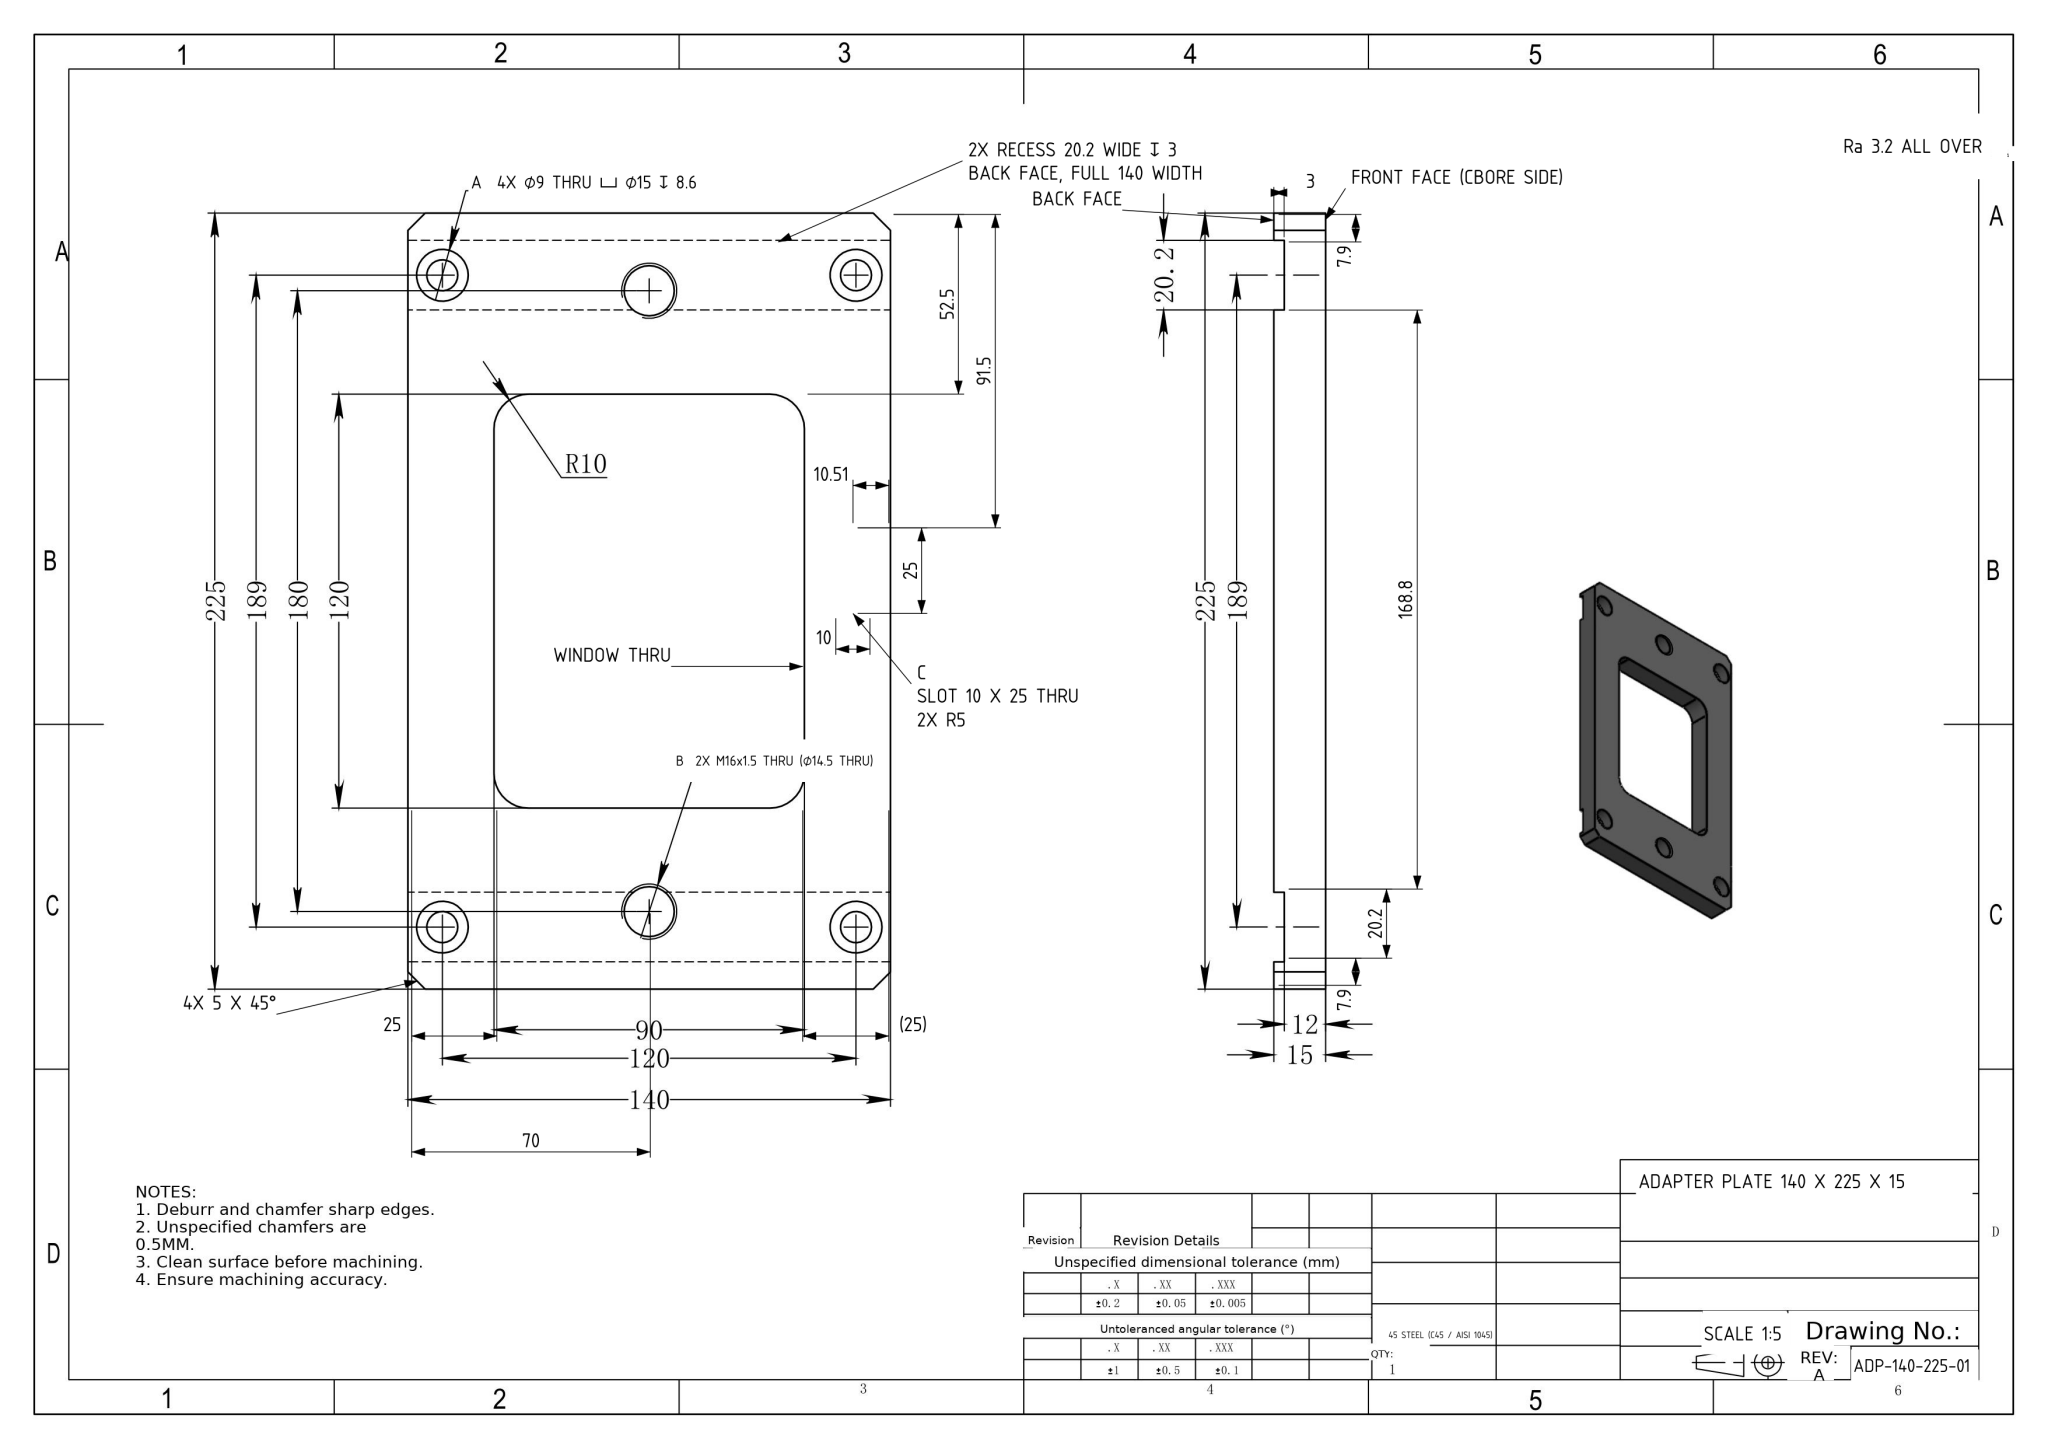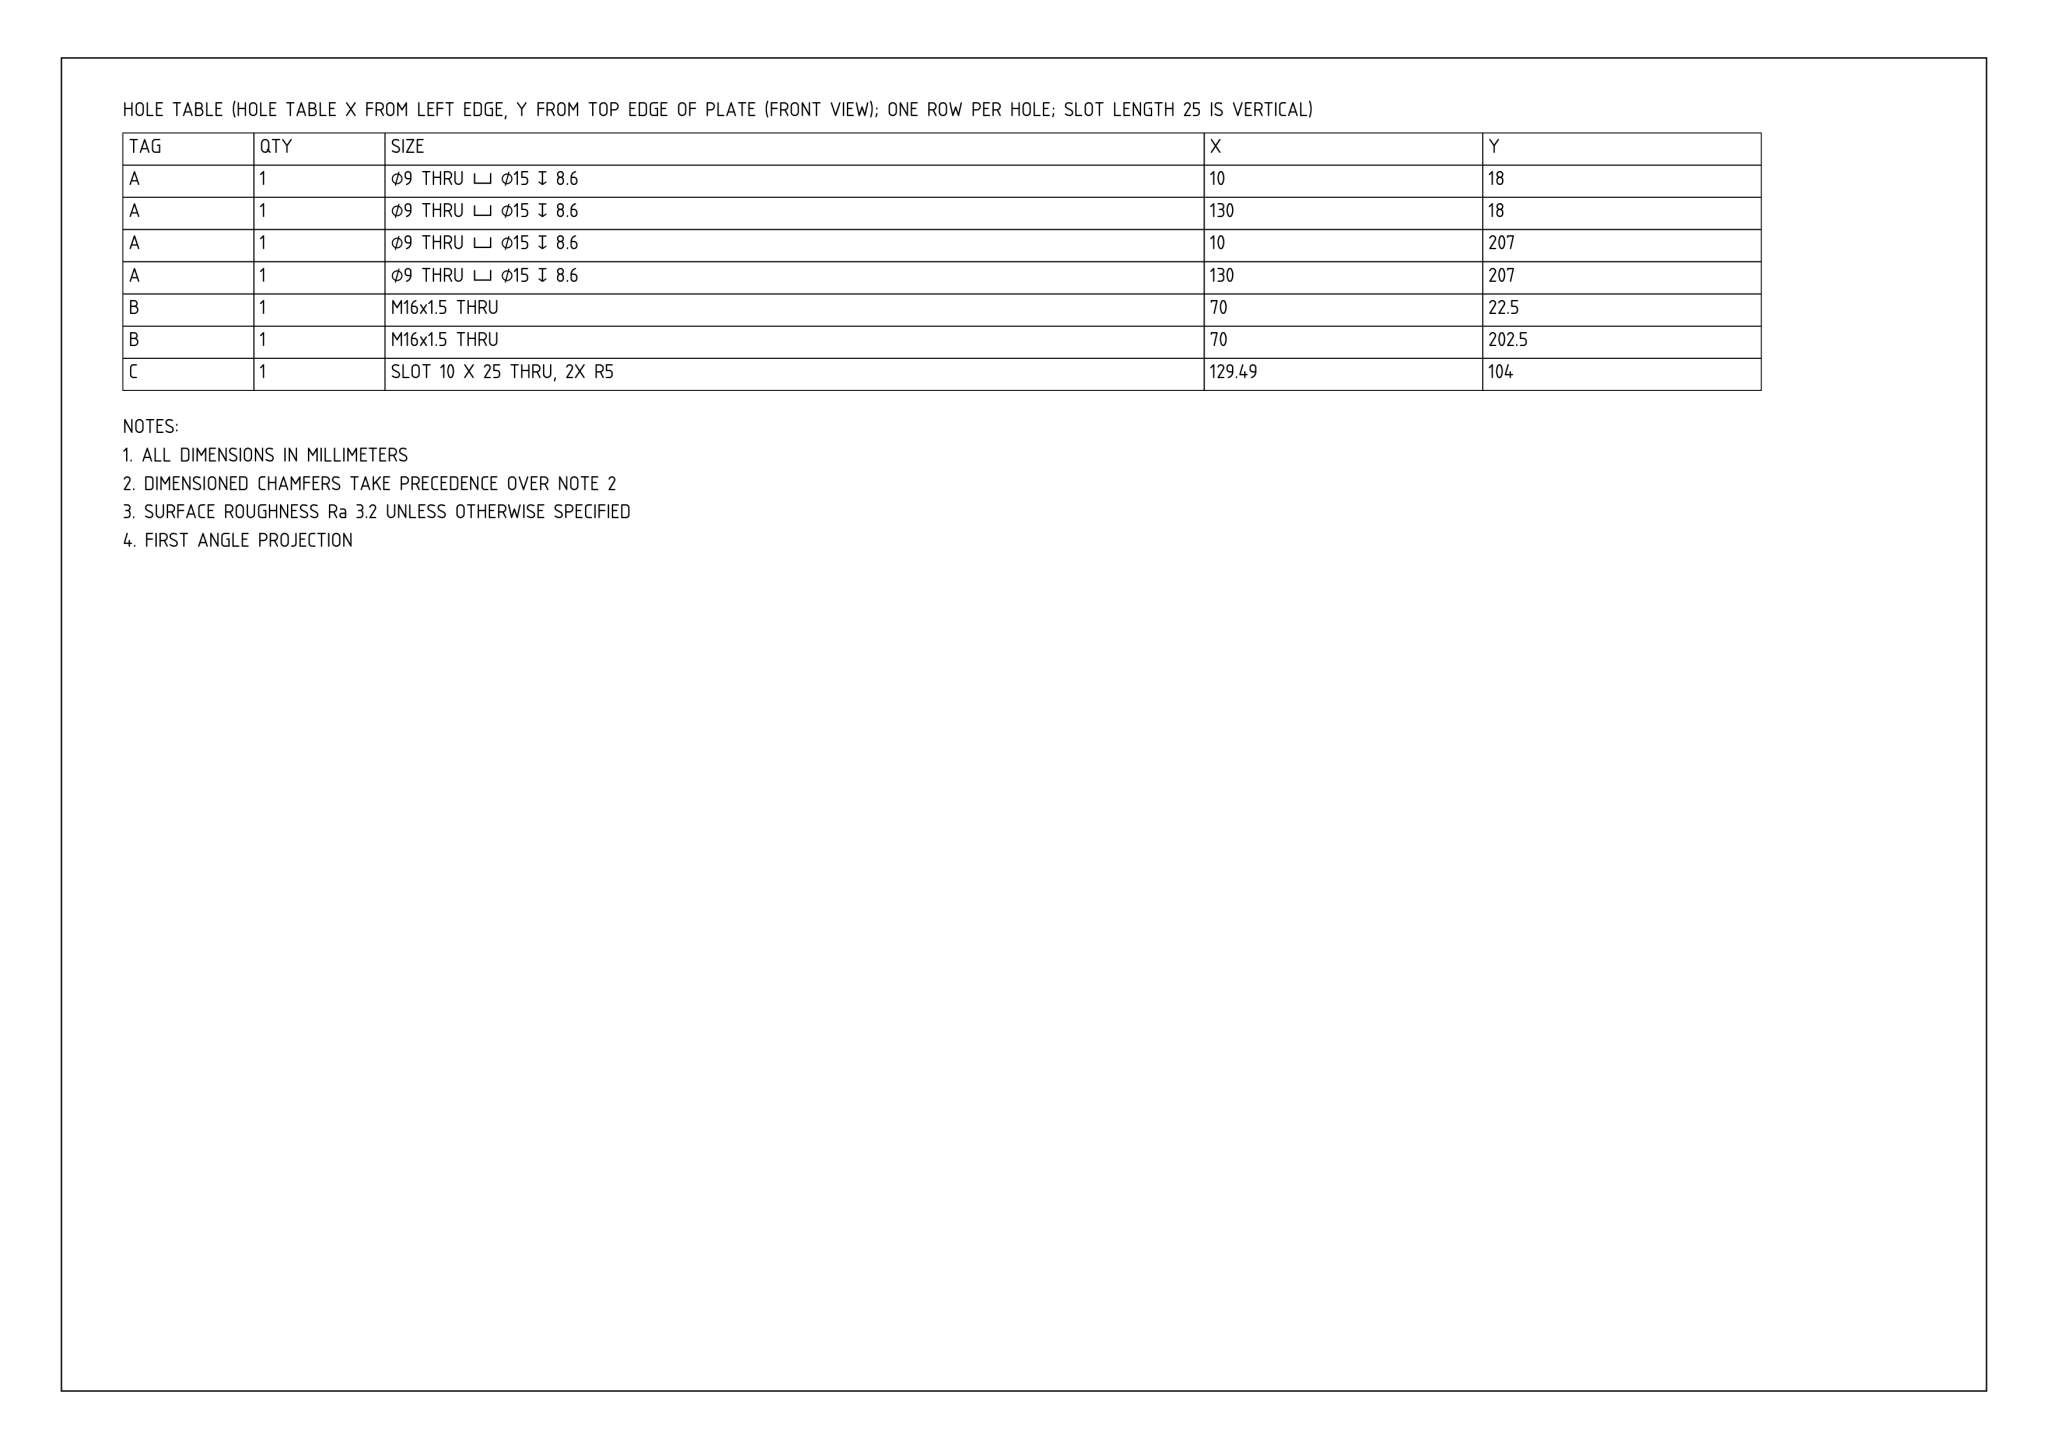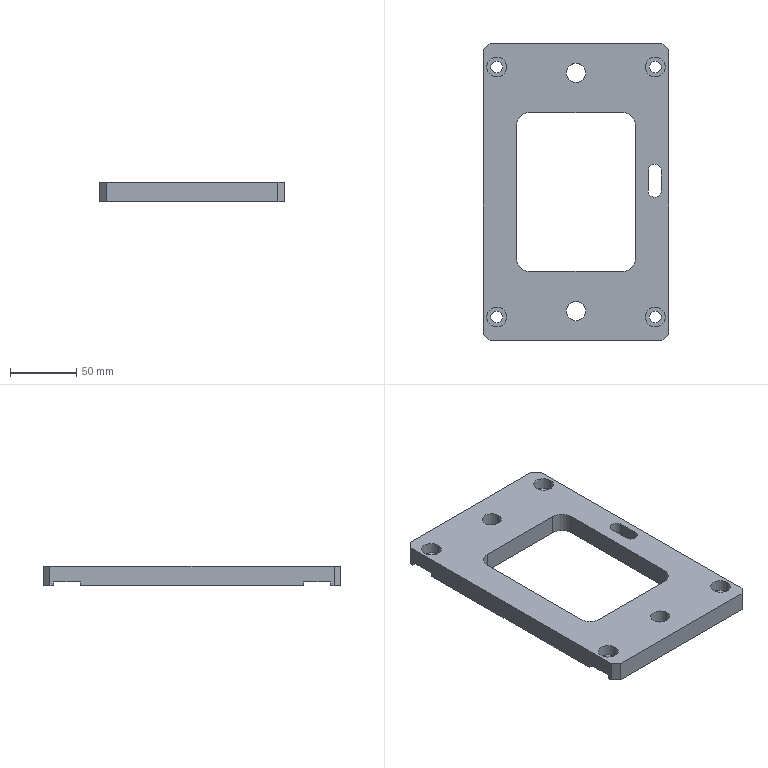Part | NX | mm | 1 solid | 56 faces | box 140 x 225 x 15 mm | volume 279672 mm3 | plane 30 | cylinder 26 | commonest cylinder face diameters 15 x8 9 x8 20 x4 14.5 x4 10 x2